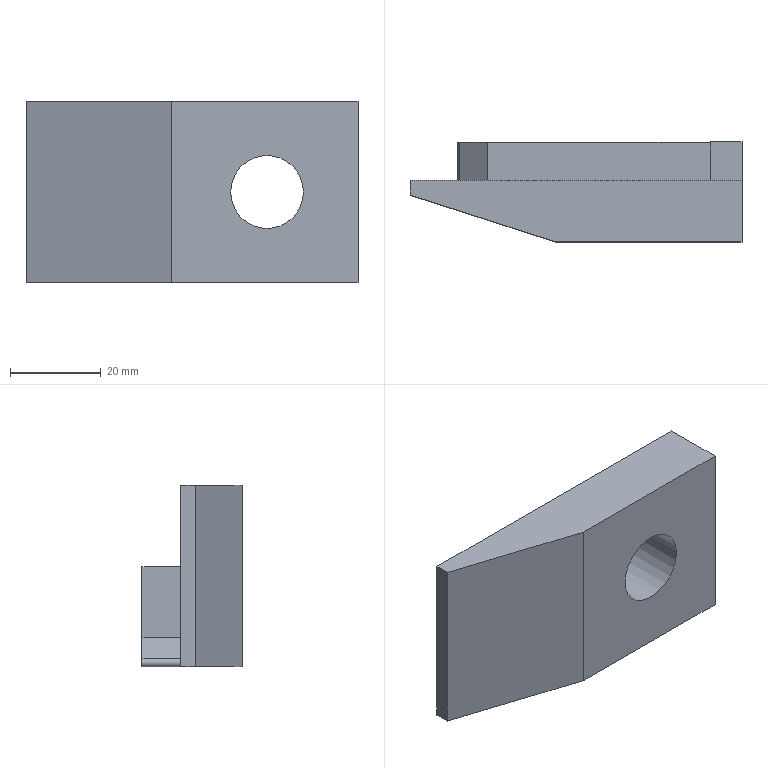Component | SolidWorks | BearingLiftingModule-1_CylinderLiftingModule-1_CHEN123-AA-28-1 | 1 solid | 15 faces | box 73 x 22 x 40 mm | volume 34379 mm3 | plane 12 | cylinder 3 | commonest cylinder face diameters 16 x2 2 x1
build123d program:
from build123d import *

# Parameters (mm, degrees)
SKETCH1_W           = 73
SKETCH1_H           = 40
BOSS_EXTRUDE1_DEPTH = 22
SKETCH2_R           = 8
CUT_EXTRUDE1_DEPTH  = 48.077
CUT_EXTRUDE2_DEPTH  = 8.5
CUT_EXTRUDE3_DEPTH  = 8.5
FILLET2_R           = 1
CUT_EXTRUDE4_DEPTH  = 59.449


with BuildPart() as part:
    # Sketch1 → Boss-Extrude1 (new body)
    with BuildSketch(Plane.XY):
        Rectangle(SKETCH1_W, SKETCH1_H)
    extrude(amount=BOSS_EXTRUDE1_DEPTH)

    # Sketch2 → Cut-Extrude1 (cut, through all)
    with BuildSketch(Plane.XY.offset(22)):
        with Locations((16.5, 0)):
            Circle(SKETCH2_R)
    extrude(amount=-CUT_EXTRUDE1_DEPTH, mode=Mode.SUBTRACT)

    # Sketch3 → Cut-Extrude2 (cut)
    with BuildSketch(Plane.XY.offset(22)):
        Polygon((-36.5, 13.5), (29.5, 13.5), (29.5, -2), (36.5, -2), (36.5, -20), (-36.5, -20), align=None)
    extrude(amount=-CUT_EXTRUDE2_DEPTH, mode=Mode.SUBTRACT)

    # Sketch4 → Cut-Extrude3 (cut)
    with BuildSketch(Plane.XY.offset(22)):
        Polygon((-36.5, 13.5), (-36.5, 26.54), (-19.469, 13.5), align=None)
    extrude(amount=-CUT_EXTRUDE3_DEPTH, mode=Mode.SUBTRACT)

    # Fillet2
    fillet2_edges = [part.edges().sort_by_distance(p)[0] for p in [
        (-27.958, 20, 17.75),
    ]]
    fillet(fillet2_edges, radius=FILLET2_R)

    # Sketch5 → Cut-Extrude4 (cut, through all)
    with BuildSketch(Plane.XZ.offset(20)):
        Polygon((-36.5, 10.253), (-4.505, 0), (-36.5, 0), align=None)
    extrude(amount=-CUT_EXTRUDE4_DEPTH, mode=Mode.SUBTRACT)


solid = part.part

# Placed as in the assembly
solid = solid.moved(Location((53.499, 21.801, 30), (-90, 0, 0)))
STEP:
#1=CARTESIAN_POINT('',(2.441,0.8583,1.181));
#2=VERTEX_POINT('',#1);
#3=CARTESIAN_POINT('',(3.071,0.8583,1.181));
#4=VERTEX_POINT('',#3);
#5=CARTESIAN_POINT('',(2.756,0.8583,1.181));
#6=DIRECTION('',(0.,1.,-0.));
#7=DIRECTION('',(1.,0.,0.));
#8=AXIS2_PLACEMENT_3D('',#5,#6,#7);
#9=CIRCLE('',#8,0.315);
#10=EDGE_CURVE('',#2,#4,#9,.T.);
#11=ORIENTED_EDGE('',*,*,#10,.F.);
#12=CARTESIAN_POINT('',(2.441,1.39,1.181));
#13=VERTEX_POINT('',#12);
#14=CARTESIAN_POINT('',(2.441,0.8583,1.181));
#15=DIRECTION('',(0.,1.,-0.));
#16=VECTOR('',#15,39.37);
#17=LINE('',#14,#16);
#18=EDGE_CURVE('',#2,#13,#17,.T.);
#19=ORIENTED_EDGE('',*,*,#18,.T.);
#20=CARTESIAN_POINT('',(3.071,1.39,1.181));
#21=VERTEX_POINT('',#20);
#22=CARTESIAN_POINT('',(2.756,1.39,1.181));
#23=DIRECTION('',(0.,1.,-0.));
#24=DIRECTION('',(-1.,0.,0.));
#25=AXIS2_PLACEMENT_3D('',#22,#23,#24);
#26=CIRCLE('',#25,0.315);
#27=EDGE_CURVE('',#13,#21,#26,.T.);
#28=ORIENTED_EDGE('',*,*,#27,.T.);
#29=CARTESIAN_POINT('',(3.071,0.8583,1.181));
#30=DIRECTION('',(0.,1.,-0.));
#31=VECTOR('',#30,39.37);
#32=LINE('',#29,#31);
#33=EDGE_CURVE('',#4,#21,#32,.T.);
#34=ORIENTED_EDGE('',*,*,#33,.F.);
#35=EDGE_LOOP('',(#11,#19,#28,#34));
#36=FACE_OUTER_BOUND('',#35,.T.);
#37=CARTESIAN_POINT('',(2.756,0.8583,1.181));
#38=DIRECTION('',(0.,1.,-0.));
#39=DIRECTION('',(1.,0.,0.));
#40=AXIS2_PLACEMENT_3D('',#37,#38,#39);
#41=CYLINDRICAL_SURFACE('',#40,0.315);
#42=ADVANCED_FACE('',(#36),#41,.F.);
#43=CARTESIAN_POINT('',(3.543,1.724,1.26));
#44=VERTEX_POINT('',#43);
#45=CARTESIAN_POINT('',(3.543,1.724,0.3937));
#46=VERTEX_POINT('',#45);
#47=CARTESIAN_POINT('',(3.543,1.724,1.969));
#48=DIRECTION('',(-0.,-0.,-1.));
#49=VECTOR('',#48,39.37);
#50=LINE('',#47,#49);
#51=EDGE_CURVE('',#44,#46,#50,.T.);
#52=ORIENTED_EDGE('',*,*,#51,.F.);
#53=CARTESIAN_POINT('',(3.543,1.39,1.26));
#54=VERTEX_POINT('',#53);
#55=CARTESIAN_POINT('',(3.543,1.39,1.26));
#56=DIRECTION('',(0.,1.,-0.));
#57=VECTOR('',#56,39.37);
#58=LINE('',#55,#57);
#59=EDGE_CURVE('',#54,#44,#58,.T.);
#60=ORIENTED_EDGE('',*,*,#59,.F.);
#61=CARTESIAN_POINT('',(3.543,1.39,1.969));
#62=VERTEX_POINT('',#61);
#63=CARTESIAN_POINT('',(3.543,1.39,1.26));
#64=DIRECTION('',(-0.,-0.,-1.));
#65=VECTOR('',#64,39.37);
#66=LINE('',#63,#65);
#67=EDGE_CURVE('',#62,#54,#66,.T.);
#68=ORIENTED_EDGE('',*,*,#67,.F.);
#69=CARTESIAN_POINT('',(3.543,0.8583,1.969));
#70=VERTEX_POINT('',#69);
#71=CARTESIAN_POINT('',(3.543,1.724,1.969));
#72=DIRECTION('',(0.,-1.,0.));
#73=VECTOR('',#72,39.37);
#74=LINE('',#71,#73);
#75=EDGE_CURVE('',#62,#70,#74,.T.);
#76=ORIENTED_EDGE('',*,*,#75,.T.);
#77=CARTESIAN_POINT('',(3.543,0.8583,0.3937));
#78=VERTEX_POINT('',#77);
#79=CARTESIAN_POINT('',(3.543,0.8583,1.969));
#80=DIRECTION('',(-0.,-0.,-1.));
#81=VECTOR('',#80,39.37);
#82=LINE('',#79,#81);
#83=EDGE_CURVE('',#70,#78,#82,.T.);
#84=ORIENTED_EDGE('',*,*,#83,.T.);
#85=CARTESIAN_POINT('',(3.543,1.724,0.3937));
#86=DIRECTION('',(0.,-1.,0.));
#87=VECTOR('',#86,39.37);
#88=LINE('',#85,#87);
#89=EDGE_CURVE('',#46,#78,#88,.T.);
#90=ORIENTED_EDGE('',*,*,#89,.F.);
#91=EDGE_LOOP('',(#52,#60,#68,#76,#84,#90));
#92=FACE_OUTER_BOUND('',#91,.T.);
#93=CARTESIAN_POINT('',(3.543,1.724,1.969));
#94=DIRECTION('',(-1.,0.,0.));
#95=DIRECTION('',(0.,1.,-0.));
#96=AXIS2_PLACEMENT_3D('',#93,#94,#95);
#97=PLANE('',#96);
#98=ADVANCED_FACE('',(#92),#97,.F.);
#99=CARTESIAN_POINT('',(1.929,0.8583,0.3937));
#100=VERTEX_POINT('',#99);
#101=CARTESIAN_POINT('',(0.6693,0.8583,0.3937));
#102=DIRECTION('',(-1.,0.,0.));
#103=VECTOR('',#102,39.37);
#104=LINE('',#101,#103);
#105=EDGE_CURVE('',#78,#100,#104,.T.);
#106=ORIENTED_EDGE('',*,*,#105,.T.);
#107=CARTESIAN_POINT('',(0.6693,1.262,0.3937));
#108=VERTEX_POINT('',#107);
#109=CARTESIAN_POINT('',(0.6693,1.262,0.3937));
#110=DIRECTION('',(-0.9523,0.3052,0.));
#111=VECTOR('',#110,39.37);
#112=LINE('',#109,#111);
#113=EDGE_CURVE('',#100,#108,#112,.T.);
#114=ORIENTED_EDGE('',*,*,#113,.T.);
#115=CARTESIAN_POINT('',(0.6693,1.39,0.3937));
#116=VERTEX_POINT('',#115);
#117=CARTESIAN_POINT('',(0.6693,1.724,0.3937));
#118=DIRECTION('',(0.,-1.,0.));
#119=VECTOR('',#118,39.37);
#120=LINE('',#117,#119);
#121=EDGE_CURVE('',#116,#108,#120,.T.);
#122=ORIENTED_EDGE('',*,*,#121,.F.);
#123=CARTESIAN_POINT('',(1.122,1.39,0.3937));
#124=VERTEX_POINT('',#123);
#125=CARTESIAN_POINT('',(0.6693,1.39,0.3937));
#126=DIRECTION('',(1.,-0.,-0.));
#127=VECTOR('',#126,39.37);
#128=LINE('',#125,#127);
#129=EDGE_CURVE('',#116,#124,#128,.T.);
#130=ORIENTED_EDGE('',*,*,#129,.T.);
#131=CARTESIAN_POINT('',(1.122,1.724,0.3937));
#132=VERTEX_POINT('',#131);
#133=CARTESIAN_POINT('',(1.122,1.724,0.3937));
#134=DIRECTION('',(0.,1.,-0.));
#135=VECTOR('',#134,39.37);
#136=LINE('',#133,#135);
#137=EDGE_CURVE('',#124,#132,#136,.T.);
#138=ORIENTED_EDGE('',*,*,#137,.T.);
#139=CARTESIAN_POINT('',(0.6693,1.724,0.3937));
#140=DIRECTION('',(-1.,0.,0.));
#141=VECTOR('',#140,39.37);
#142=LINE('',#139,#141);
#143=EDGE_CURVE('',#46,#132,#142,.T.);
#144=ORIENTED_EDGE('',*,*,#143,.F.);
#145=ORIENTED_EDGE('',*,*,#89,.T.);
#146=EDGE_LOOP('',(#106,#114,#122,#130,#138,#144,#145));
#147=FACE_OUTER_BOUND('',#146,.T.);
#148=CARTESIAN_POINT('',(0.6693,1.724,0.3937));
#149=DIRECTION('',(0.,0.,1.));
#150=DIRECTION('',(0.,-1.,0.));
#151=AXIS2_PLACEMENT_3D('',#148,#149,#150);
#152=PLANE('',#151);
#153=ADVANCED_FACE('',(#147),#152,.F.);
#154=ORIENTED_EDGE('',*,*,#121,.T.);
#155=CARTESIAN_POINT('',(0.6693,1.262,1.969));
#156=VERTEX_POINT('',#155);
#157=CARTESIAN_POINT('',(0.6693,1.262,0.3937));
#158=DIRECTION('',(0.,0.,1.));
#159=VECTOR('',#158,39.37);
#160=LINE('',#157,#159);
#161=EDGE_CURVE('',#108,#156,#160,.T.);
#162=ORIENTED_EDGE('',*,*,#161,.T.);
#163=CARTESIAN_POINT('',(0.6693,1.39,1.969));
#164=VERTEX_POINT('',#163);
#165=CARTESIAN_POINT('',(0.6693,1.724,1.969));
#166=DIRECTION('',(0.,-1.,0.));
#167=VECTOR('',#166,39.37);
#168=LINE('',#165,#167);
#169=EDGE_CURVE('',#164,#156,#168,.T.);
#170=ORIENTED_EDGE('',*,*,#169,.F.);
#171=CARTESIAN_POINT('',(0.6693,1.39,1.969));
#172=DIRECTION('',(0.,0.,1.));
#173=VECTOR('',#172,39.37);
#174=LINE('',#171,#173);
#175=EDGE_CURVE('',#116,#164,#174,.T.);
#176=ORIENTED_EDGE('',*,*,#175,.F.);
#177=EDGE_LOOP('',(#154,#162,#170,#176));
#178=FACE_OUTER_BOUND('',#177,.T.);
#179=CARTESIAN_POINT('',(0.6693,1.724,1.969));
#180=DIRECTION('',(1.,-0.,-0.));
#181=DIRECTION('',(0.,-1.,0.));
#182=AXIS2_PLACEMENT_3D('',#179,#180,#181);
#183=PLANE('',#182);
#184=ADVANCED_FACE('',(#178),#183,.F.);
#185=ORIENTED_EDGE('',*,*,#169,.T.);
#186=CARTESIAN_POINT('',(1.929,0.8583,1.969));
#187=VERTEX_POINT('',#186);
#188=CARTESIAN_POINT('',(0.6693,1.262,1.969));
#189=DIRECTION('',(-0.9523,0.3052,0.));
#190=VECTOR('',#189,39.37);
#191=LINE('',#188,#190);
#192=EDGE_CURVE('',#187,#156,#191,.T.);
#193=ORIENTED_EDGE('',*,*,#192,.F.);
#194=CARTESIAN_POINT('',(0.6693,0.8583,1.969));
#195=DIRECTION('',(1.,-0.,-0.));
#196=VECTOR('',#195,39.37);
#197=LINE('',#194,#196);
#198=EDGE_CURVE('',#187,#70,#197,.T.);
#199=ORIENTED_EDGE('',*,*,#198,.T.);
#200=ORIENTED_EDGE('',*,*,#75,.F.);
#201=CARTESIAN_POINT('',(3.543,1.39,1.969));
#202=DIRECTION('',(1.,-0.,-0.));
#203=VECTOR('',#202,39.37);
#204=LINE('',#201,#203);
#205=EDGE_CURVE('',#164,#62,#204,.T.);
#206=ORIENTED_EDGE('',*,*,#205,.F.);
#207=EDGE_LOOP('',(#185,#193,#199,#200,#206));
#208=FACE_OUTER_BOUND('',#207,.T.);
#209=CARTESIAN_POINT('',(0.6693,1.724,1.969));
#210=DIRECTION('',(-0.,-0.,-1.));
#211=DIRECTION('',(0.,1.,-0.));
#212=AXIS2_PLACEMENT_3D('',#209,#210,#211);
#213=PLANE('',#212);
#214=ADVANCED_FACE('',(#208),#213,.F.);
#215=ORIENTED_EDGE('',*,*,#143,.T.);
#216=CARTESIAN_POINT('',(1.098,1.724,0.4643));
#217=VERTEX_POINT('',#216);
#218=CARTESIAN_POINT('',(1.122,1.724,0.4331));
#219=DIRECTION('',(0.,1.,-0.));
#220=DIRECTION('',(-1.,0.,0.));
#221=AXIS2_PLACEMENT_3D('',#218,#219,#220);
#222=CIRCLE('',#221,0.03937);
#223=EDGE_CURVE('',#132,#217,#222,.T.);
#224=ORIENTED_EDGE('',*,*,#223,.T.);
#225=CARTESIAN_POINT('',(1.34,1.724,0.6496));
#226=VERTEX_POINT('',#225);
#227=CARTESIAN_POINT('',(0.6693,1.724,0.1362));
#228=DIRECTION('',(-0.794,-0.,-0.6079));
#229=VECTOR('',#228,39.37);
#230=LINE('',#227,#229);
#231=EDGE_CURVE('',#226,#217,#230,.T.);
#232=ORIENTED_EDGE('',*,*,#231,.F.);
#233=CARTESIAN_POINT('',(3.268,1.724,0.6496));
#234=VERTEX_POINT('',#233);
#235=CARTESIAN_POINT('',(0.6693,1.724,0.6496));
#236=DIRECTION('',(-1.,0.,0.));
#237=VECTOR('',#236,39.37);
#238=LINE('',#235,#237);
#239=EDGE_CURVE('',#234,#226,#238,.T.);
#240=ORIENTED_EDGE('',*,*,#239,.F.);
#241=CARTESIAN_POINT('',(3.268,1.724,1.26));
#242=VERTEX_POINT('',#241);
#243=CARTESIAN_POINT('',(3.268,1.724,0.6496));
#244=DIRECTION('',(-0.,-0.,-1.));
#245=VECTOR('',#244,39.37);
#246=LINE('',#243,#245);
#247=EDGE_CURVE('',#242,#234,#246,.T.);
#248=ORIENTED_EDGE('',*,*,#247,.F.);
#249=CARTESIAN_POINT('',(3.268,1.724,1.26));
#250=DIRECTION('',(-1.,0.,0.));
#251=VECTOR('',#250,39.37);
#252=LINE('',#249,#251);
#253=EDGE_CURVE('',#44,#242,#252,.T.);
#254=ORIENTED_EDGE('',*,*,#253,.F.);
#255=ORIENTED_EDGE('',*,*,#51,.T.);
#256=EDGE_LOOP('',(#215,#224,#232,#240,#248,#254,#255));
#257=FACE_OUTER_BOUND('',#256,.T.);
#258=CARTESIAN_POINT('',(2.106,1.724,1.181));
#259=DIRECTION('',(0.,-1.,0.));
#260=DIRECTION('',(-1.,0.,0.));
#261=AXIS2_PLACEMENT_3D('',#258,#259,#260);
#262=PLANE('',#261);
#263=ADVANCED_FACE('',(#257),#262,.F.);
#264=CARTESIAN_POINT('',(1.929,0.8583,0.3937));
#265=DIRECTION('',(0.,0.,1.));
#266=VECTOR('',#265,39.37);
#267=LINE('',#264,#266);
#268=EDGE_CURVE('',#100,#187,#267,.T.);
#269=ORIENTED_EDGE('',*,*,#268,.F.);
#270=ORIENTED_EDGE('',*,*,#105,.F.);
#271=ORIENTED_EDGE('',*,*,#83,.F.);
#272=ORIENTED_EDGE('',*,*,#198,.F.);
#273=EDGE_LOOP('',(#269,#270,#271,#272));
#274=FACE_OUTER_BOUND('',#273,.T.);
#275=CARTESIAN_POINT('',(2.756,0.8583,1.181));
#276=DIRECTION('',(0.,1.,-0.));
#277=DIRECTION('',(1.,0.,0.));
#278=AXIS2_PLACEMENT_3D('',#275,#276,#277);
#279=CIRCLE('',#278,0.315);
#280=EDGE_CURVE('',#4,#2,#279,.T.);
#281=ORIENTED_EDGE('',*,*,#280,.T.);
#282=ORIENTED_EDGE('',*,*,#10,.T.);
#283=EDGE_LOOP('',(#281,#282));
#284=FACE_BOUND('',#283,.T.);
#285=CARTESIAN_POINT('',(2.106,0.8583,1.181));
#286=DIRECTION('',(0.,-1.,0.));
#287=DIRECTION('',(-1.,0.,0.));
#288=AXIS2_PLACEMENT_3D('',#285,#286,#287);
#289=PLANE('',#288);
#290=ADVANCED_FACE('',(#274,#284),#289,.T.);
#291=ORIENTED_EDGE('',*,*,#18,.F.);
#292=ORIENTED_EDGE('',*,*,#280,.F.);
#293=ORIENTED_EDGE('',*,*,#33,.T.);
#294=CARTESIAN_POINT('',(2.756,1.39,1.181));
#295=DIRECTION('',(0.,1.,-0.));
#296=DIRECTION('',(-1.,0.,0.));
#297=AXIS2_PLACEMENT_3D('',#294,#295,#296);
#298=CIRCLE('',#297,0.315);
#299=EDGE_CURVE('',#21,#13,#298,.T.);
#300=ORIENTED_EDGE('',*,*,#299,.T.);
#301=EDGE_LOOP('',(#291,#292,#293,#300));
#302=FACE_OUTER_BOUND('',#301,.T.);
#303=CARTESIAN_POINT('',(2.756,0.8583,1.181));
#304=DIRECTION('',(0.,1.,-0.));
#305=DIRECTION('',(1.,0.,0.));
#306=AXIS2_PLACEMENT_3D('',#303,#304,#305);
#307=CYLINDRICAL_SURFACE('',#306,0.315);
#308=ADVANCED_FACE('',(#302),#307,.F.);
#309=ORIENTED_EDGE('',*,*,#175,.T.);
#310=ORIENTED_EDGE('',*,*,#205,.T.);
#311=ORIENTED_EDGE('',*,*,#67,.T.);
#312=CARTESIAN_POINT('',(3.268,1.39,1.26));
#313=VERTEX_POINT('',#312);
#314=CARTESIAN_POINT('',(3.268,1.39,1.26));
#315=DIRECTION('',(-1.,0.,0.));
#316=VECTOR('',#315,39.37);
#317=LINE('',#314,#316);
#318=EDGE_CURVE('',#54,#313,#317,.T.);
#319=ORIENTED_EDGE('',*,*,#318,.T.);
#320=CARTESIAN_POINT('',(3.268,1.39,0.6496));
#321=VERTEX_POINT('',#320);
#322=CARTESIAN_POINT('',(3.268,1.39,0.6496));
#323=DIRECTION('',(-0.,-0.,-1.));
#324=VECTOR('',#323,39.37);
#325=LINE('',#322,#324);
#326=EDGE_CURVE('',#313,#321,#325,.T.);
#327=ORIENTED_EDGE('',*,*,#326,.T.);
#328=CARTESIAN_POINT('',(1.34,1.39,0.6496));
#329=VERTEX_POINT('',#328);
#330=CARTESIAN_POINT('',(0.6693,1.39,0.6496));
#331=DIRECTION('',(-1.,0.,0.));
#332=VECTOR('',#331,39.37);
#333=LINE('',#330,#332);
#334=EDGE_CURVE('',#321,#329,#333,.T.);
#335=ORIENTED_EDGE('',*,*,#334,.T.);
#336=CARTESIAN_POINT('',(1.098,1.39,0.4643));
#337=VERTEX_POINT('',#336);
#338=CARTESIAN_POINT('',(0.6693,1.39,0.1362));
#339=DIRECTION('',(-0.794,-0.,-0.6079));
#340=VECTOR('',#339,39.37);
#341=LINE('',#338,#340);
#342=EDGE_CURVE('',#329,#337,#341,.T.);
#343=ORIENTED_EDGE('',*,*,#342,.T.);
#344=CARTESIAN_POINT('',(1.122,1.39,0.4331));
#345=DIRECTION('',(0.,-1.,0.));
#346=DIRECTION('',(-1.,0.,0.));
#347=AXIS2_PLACEMENT_3D('',#344,#345,#346);
#348=CIRCLE('',#347,0.03937);
#349=EDGE_CURVE('',#337,#124,#348,.T.);
#350=ORIENTED_EDGE('',*,*,#349,.T.);
#351=ORIENTED_EDGE('',*,*,#129,.F.);
#352=EDGE_LOOP('',(#309,#310,#311,#319,#327,#335,#343,#350,#351));
#353=FACE_OUTER_BOUND('',#352,.T.);
#354=ORIENTED_EDGE('',*,*,#299,.F.);
#355=ORIENTED_EDGE('',*,*,#27,.F.);
#356=EDGE_LOOP('',(#354,#355));
#357=FACE_BOUND('',#356,.T.);
#358=CARTESIAN_POINT('',(2.106,1.39,1.181));
#359=DIRECTION('',(0.,-1.,0.));
#360=DIRECTION('',(-1.,0.,0.));
#361=AXIS2_PLACEMENT_3D('',#358,#359,#360);
#362=PLANE('',#361);
#363=ADVANCED_FACE('',(#353,#357),#362,.F.);
#364=ORIENTED_EDGE('',*,*,#239,.T.);
#365=CARTESIAN_POINT('',(1.34,1.39,0.6496));
#366=DIRECTION('',(0.,1.,-0.));
#367=VECTOR('',#366,39.37);
#368=LINE('',#365,#367);
#369=EDGE_CURVE('',#329,#226,#368,.T.);
#370=ORIENTED_EDGE('',*,*,#369,.F.);
#371=ORIENTED_EDGE('',*,*,#334,.F.);
#372=CARTESIAN_POINT('',(3.268,1.39,0.6496));
#373=DIRECTION('',(0.,1.,-0.));
#374=VECTOR('',#373,39.37);
#375=LINE('',#372,#374);
#376=EDGE_CURVE('',#321,#234,#375,.T.);
#377=ORIENTED_EDGE('',*,*,#376,.T.);
#378=EDGE_LOOP('',(#364,#370,#371,#377));
#379=FACE_OUTER_BOUND('',#378,.T.);
#380=CARTESIAN_POINT('',(0.6693,1.39,0.6496));
#381=DIRECTION('',(-0.,-0.,-1.));
#382=DIRECTION('',(0.,1.,-0.));
#383=AXIS2_PLACEMENT_3D('',#380,#381,#382);
#384=PLANE('',#383);
#385=ADVANCED_FACE('',(#379),#384,.F.);
#386=ORIENTED_EDGE('',*,*,#247,.T.);
#387=ORIENTED_EDGE('',*,*,#376,.F.);
#388=ORIENTED_EDGE('',*,*,#326,.F.);
#389=CARTESIAN_POINT('',(3.268,1.39,1.26));
#390=DIRECTION('',(0.,1.,-0.));
#391=VECTOR('',#390,39.37);
#392=LINE('',#389,#391);
#393=EDGE_CURVE('',#313,#242,#392,.T.);
#394=ORIENTED_EDGE('',*,*,#393,.T.);
#395=EDGE_LOOP('',(#386,#387,#388,#394));
#396=FACE_OUTER_BOUND('',#395,.T.);
#397=CARTESIAN_POINT('',(3.268,1.39,0.6496));
#398=DIRECTION('',(1.,-0.,-0.));
#399=DIRECTION('',(-0.,-0.,-1.));
#400=AXIS2_PLACEMENT_3D('',#397,#398,#399);
#401=PLANE('',#400);
#402=ADVANCED_FACE('',(#396),#401,.F.);
#403=ORIENTED_EDGE('',*,*,#253,.T.);
#404=ORIENTED_EDGE('',*,*,#393,.F.);
#405=ORIENTED_EDGE('',*,*,#318,.F.);
#406=ORIENTED_EDGE('',*,*,#59,.T.);
#407=EDGE_LOOP('',(#403,#404,#405,#406));
#408=FACE_OUTER_BOUND('',#407,.T.);
#409=CARTESIAN_POINT('',(3.268,1.39,1.26));
#410=DIRECTION('',(-0.,-0.,-1.));
#411=DIRECTION('',(0.,1.,-0.));
#412=AXIS2_PLACEMENT_3D('',#409,#410,#411);
#413=PLANE('',#412);
#414=ADVANCED_FACE('',(#408),#413,.F.);
#415=ORIENTED_EDGE('',*,*,#231,.T.);
#416=CARTESIAN_POINT('',(1.098,1.39,0.4643));
#417=DIRECTION('',(0.,-1.,0.));
#418=VECTOR('',#417,39.37);
#419=LINE('',#416,#418);
#420=EDGE_CURVE('',#217,#337,#419,.T.);
#421=ORIENTED_EDGE('',*,*,#420,.T.);
#422=ORIENTED_EDGE('',*,*,#342,.F.);
#423=ORIENTED_EDGE('',*,*,#369,.T.);
#424=EDGE_LOOP('',(#415,#421,#422,#423));
#425=FACE_OUTER_BOUND('',#424,.T.);
#426=CARTESIAN_POINT('',(0.6693,1.39,0.1362));
#427=DIRECTION('',(0.6079,-0.,-0.794));
#428=DIRECTION('',(-0.794,-0.,-0.6079));
#429=AXIS2_PLACEMENT_3D('',#426,#427,#428);
#430=PLANE('',#429);
#431=ADVANCED_FACE('',(#425),#430,.F.);
#432=ORIENTED_EDGE('',*,*,#349,.F.);
#433=ORIENTED_EDGE('',*,*,#420,.F.);
#434=ORIENTED_EDGE('',*,*,#223,.F.);
#435=ORIENTED_EDGE('',*,*,#137,.F.);
#436=EDGE_LOOP('',(#432,#433,#434,#435));
#437=FACE_OUTER_BOUND('',#436,.T.);
#438=CARTESIAN_POINT('',(1.122,1.724,0.4331));
#439=DIRECTION('',(0.,1.,-0.));
#440=DIRECTION('',(1.,0.,0.));
#441=AXIS2_PLACEMENT_3D('',#438,#439,#440);
#442=CYLINDRICAL_SURFACE('',#441,0.03937);
#443=ADVANCED_FACE('',(#437),#442,.T.);
#444=ORIENTED_EDGE('',*,*,#192,.T.);
#445=ORIENTED_EDGE('',*,*,#161,.F.);
#446=ORIENTED_EDGE('',*,*,#113,.F.);
#447=ORIENTED_EDGE('',*,*,#268,.T.);
#448=EDGE_LOOP('',(#444,#445,#446,#447));
#449=FACE_OUTER_BOUND('',#448,.T.);
#450=CARTESIAN_POINT('',(0.6693,1.262,0.3937));
#451=DIRECTION('',(0.3052,0.9523,-0.));
#452=DIRECTION('',(0.9523,-0.3052,-0.));
#453=AXIS2_PLACEMENT_3D('',#450,#451,#452);
#454=PLANE('',#453);
#455=ADVANCED_FACE('',(#449),#454,.F.);
#456=CLOSED_SHELL('',(#42,#98,#153,#184,#214,#263,#290,#308,#363,#385,#402,#414,#431,#443,#455));
#457=MANIFOLD_SOLID_BREP('',#456);
#458=CARTESIAN_POINT('',(0.,0.,0.));
#459=DIRECTION('',(0.,0.,1.));
#460=DIRECTION('',(1.,0.,0.));
#461=AXIS2_PLACEMENT_3D('',#458,#459,#460);
#462=(LENGTH_UNIT()NAMED_UNIT(*)SI_UNIT($,.METRE.));
#463=LENGTH_MEASURE_WITH_UNIT(LENGTH_MEASURE(0.0254),#462);
#464=DIMENSIONAL_EXPONENTS(1.,0.,0.,0.,0.,0.,0.);
#465=(CONVERSION_BASED_UNIT('',#463)LENGTH_UNIT()NAMED_UNIT(#464));
#466=UNCERTAINTY_MEASURE_WITH_UNIT(LENGTH_MEASURE(0.00001),#465,'','');
#467=(NAMED_UNIT(*)PLANE_ANGLE_UNIT()SI_UNIT($,.RADIAN.));
#468=(NAMED_UNIT(*)SI_UNIT($,.STERADIAN.)SOLID_ANGLE_UNIT());
#469=(GEOMETRIC_REPRESENTATION_CONTEXT(3)GLOBAL_UNCERTAINTY_ASSIGNED_CONTEXT((#466))GLOBAL_UNIT_ASSIGNED_CONTEXT((#465,#467,#468))REPRESENTATION_CONTEXT('',''));
#470=ADVANCED_BREP_SHAPE_REPRESENTATION('',(#457,#461),#469);
#471=COLOUR_RGB('',0.7922,0.8196,0.9333);
#472=FILL_AREA_STYLE_COLOUR('',#471);
#473=FILL_AREA_STYLE('',(#472));
#474=SURFACE_STYLE_FILL_AREA(#473);
#475=SURFACE_SIDE_STYLE('',(#474));
#476=SURFACE_STYLE_USAGE(.BOTH.,#475);
#477=PRESENTATION_STYLE_ASSIGNMENT((#476));
#478=STYLED_ITEM('',(#477),#457);
#479=PRESENTATION_LAYER_ASSIGNMENT('','',(#478));
#480=(LENGTH_UNIT()NAMED_UNIT(*)SI_UNIT($,.METRE.));
#481=LENGTH_MEASURE_WITH_UNIT(LENGTH_MEASURE(0.0254),#480);
#482=DIMENSIONAL_EXPONENTS(1.,0.,0.,0.,0.,0.,0.);
#483=(CONVERSION_BASED_UNIT('',#481)LENGTH_UNIT()NAMED_UNIT(#482));
#484=UNCERTAINTY_MEASURE_WITH_UNIT(LENGTH_MEASURE(0.00001),#483,'','');
#485=(NAMED_UNIT(*)PLANE_ANGLE_UNIT()SI_UNIT($,.RADIAN.));
#486=(NAMED_UNIT(*)SI_UNIT($,.STERADIAN.)SOLID_ANGLE_UNIT());
#487=(GEOMETRIC_REPRESENTATION_CONTEXT(3)GLOBAL_UNCERTAINTY_ASSIGNED_CONTEXT((#484))GLOBAL_UNIT_ASSIGNED_CONTEXT((#483,#485,#486))REPRESENTATION_CONTEXT('',''));
#488=MECHANICAL_DESIGN_GEOMETRIC_PRESENTATION_REPRESENTATION('',(#478),#487);